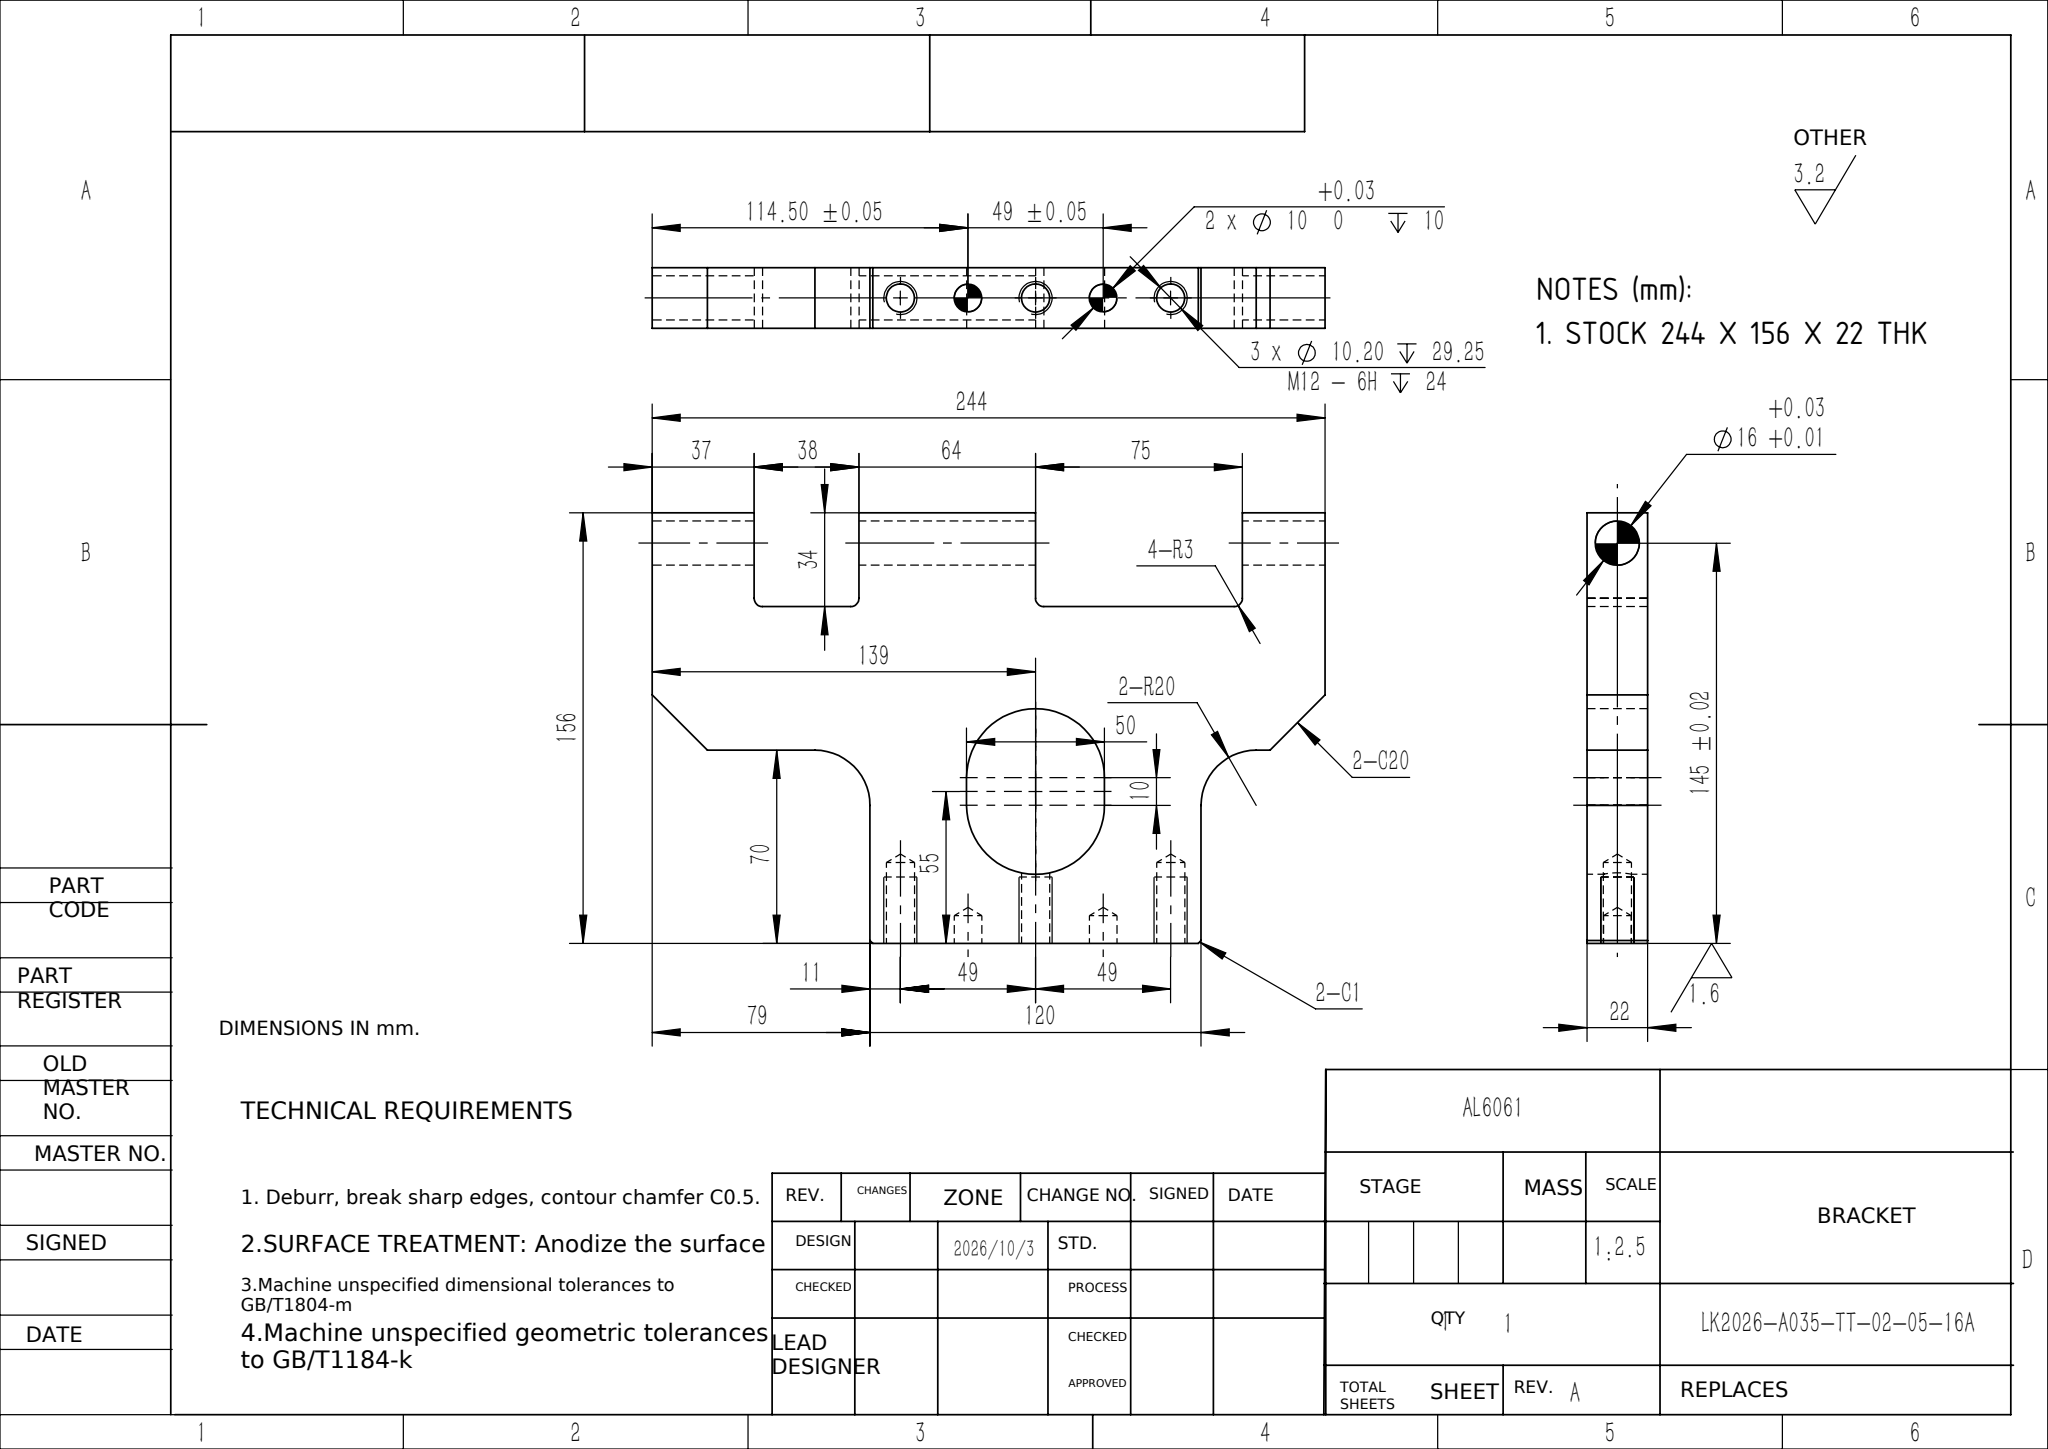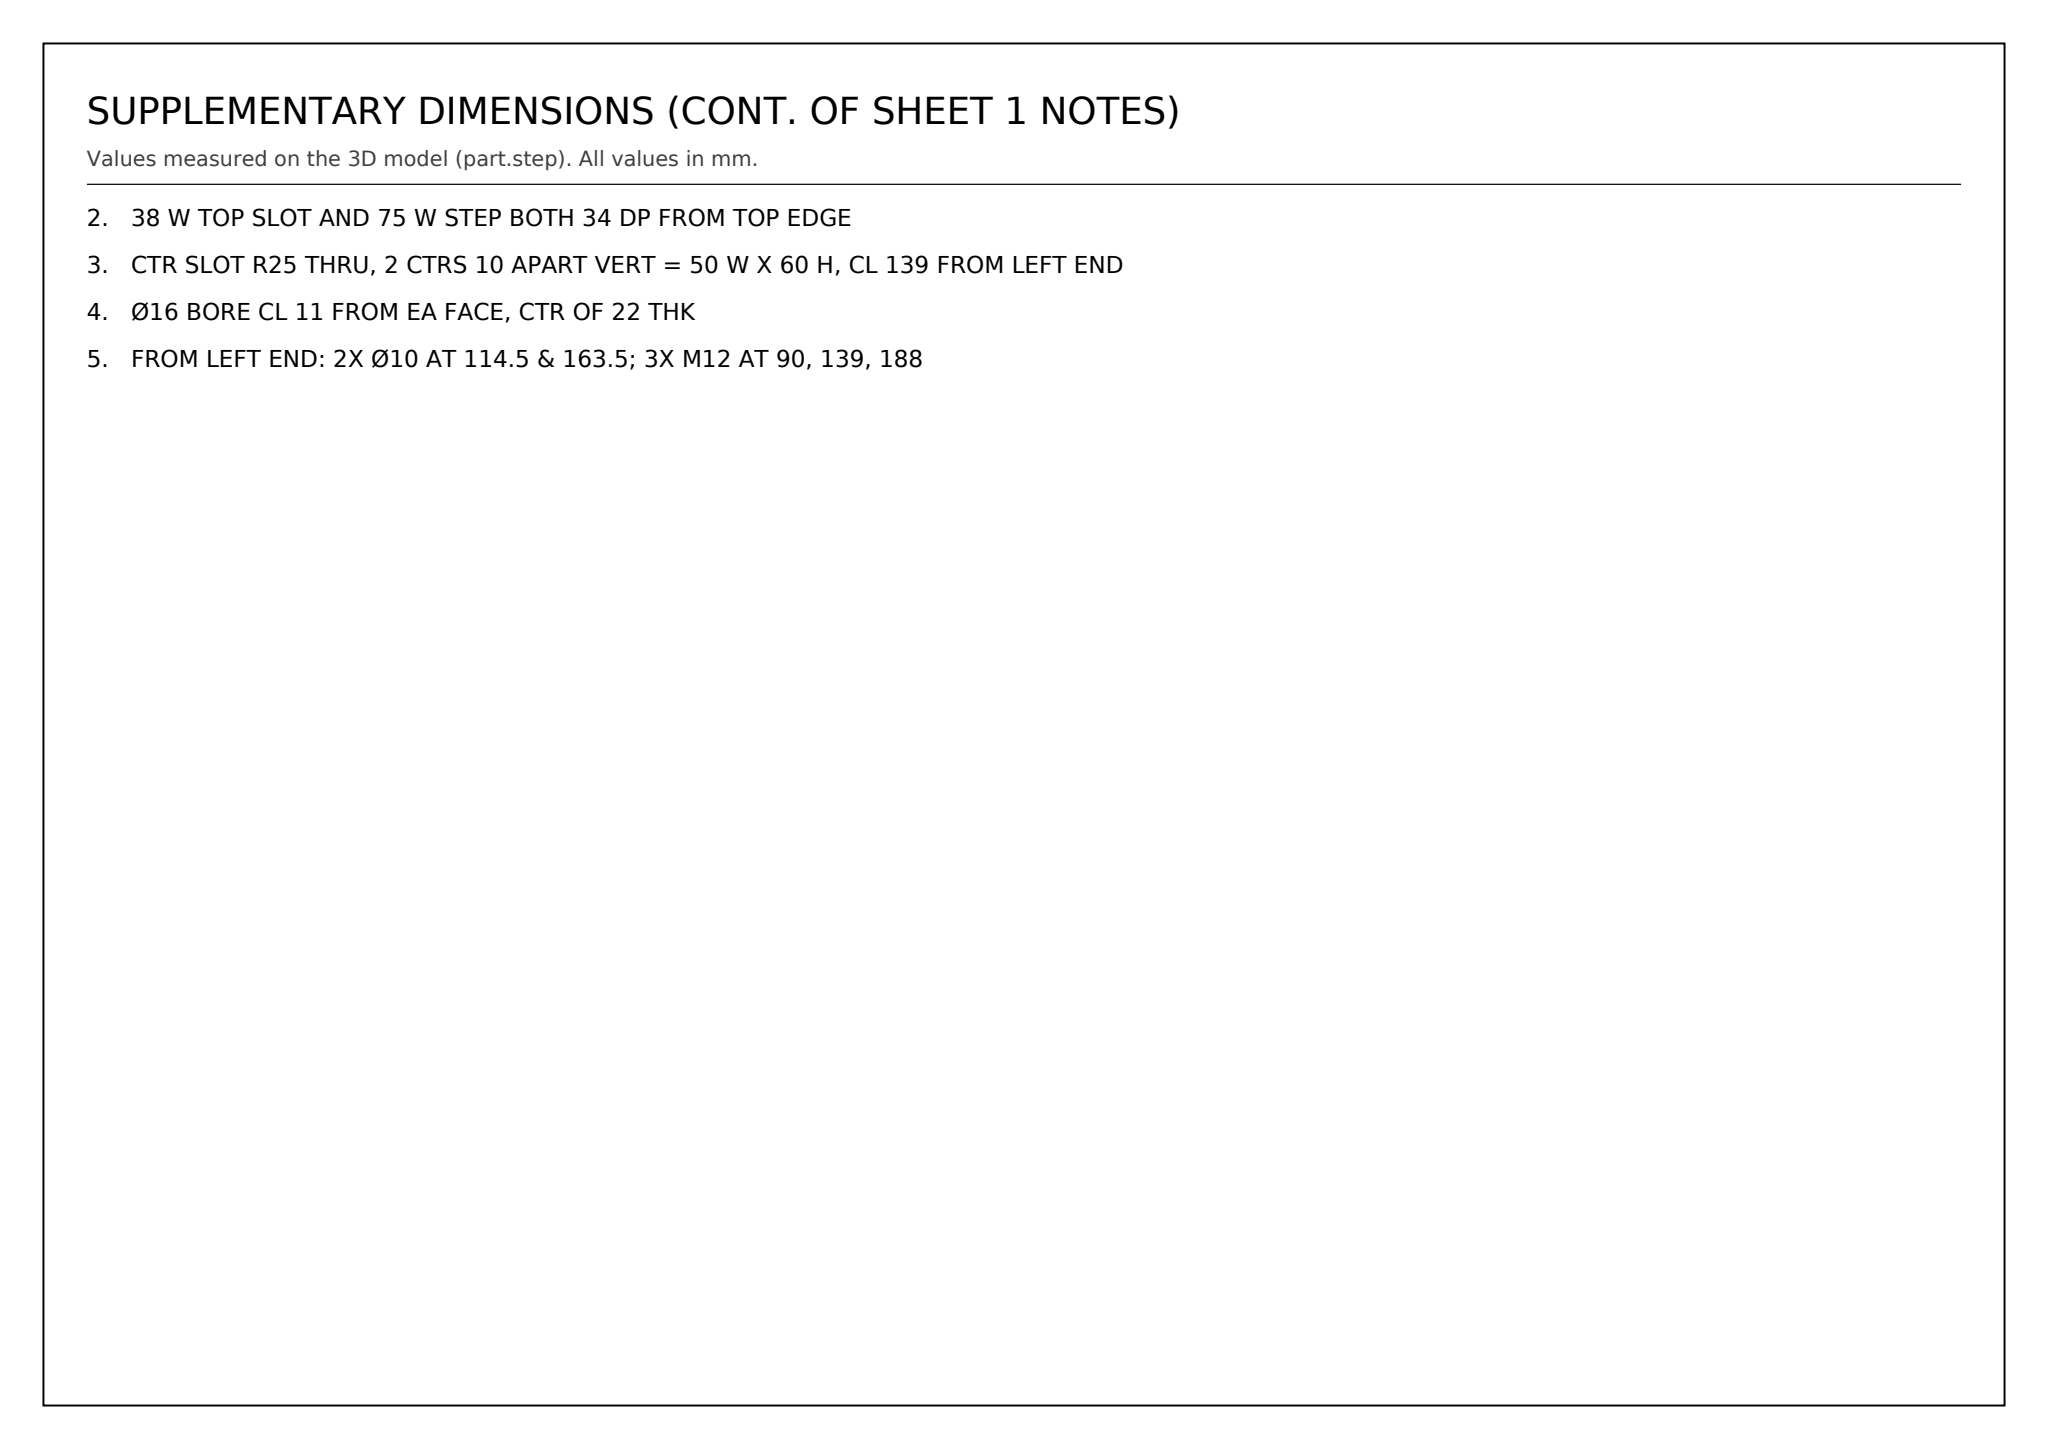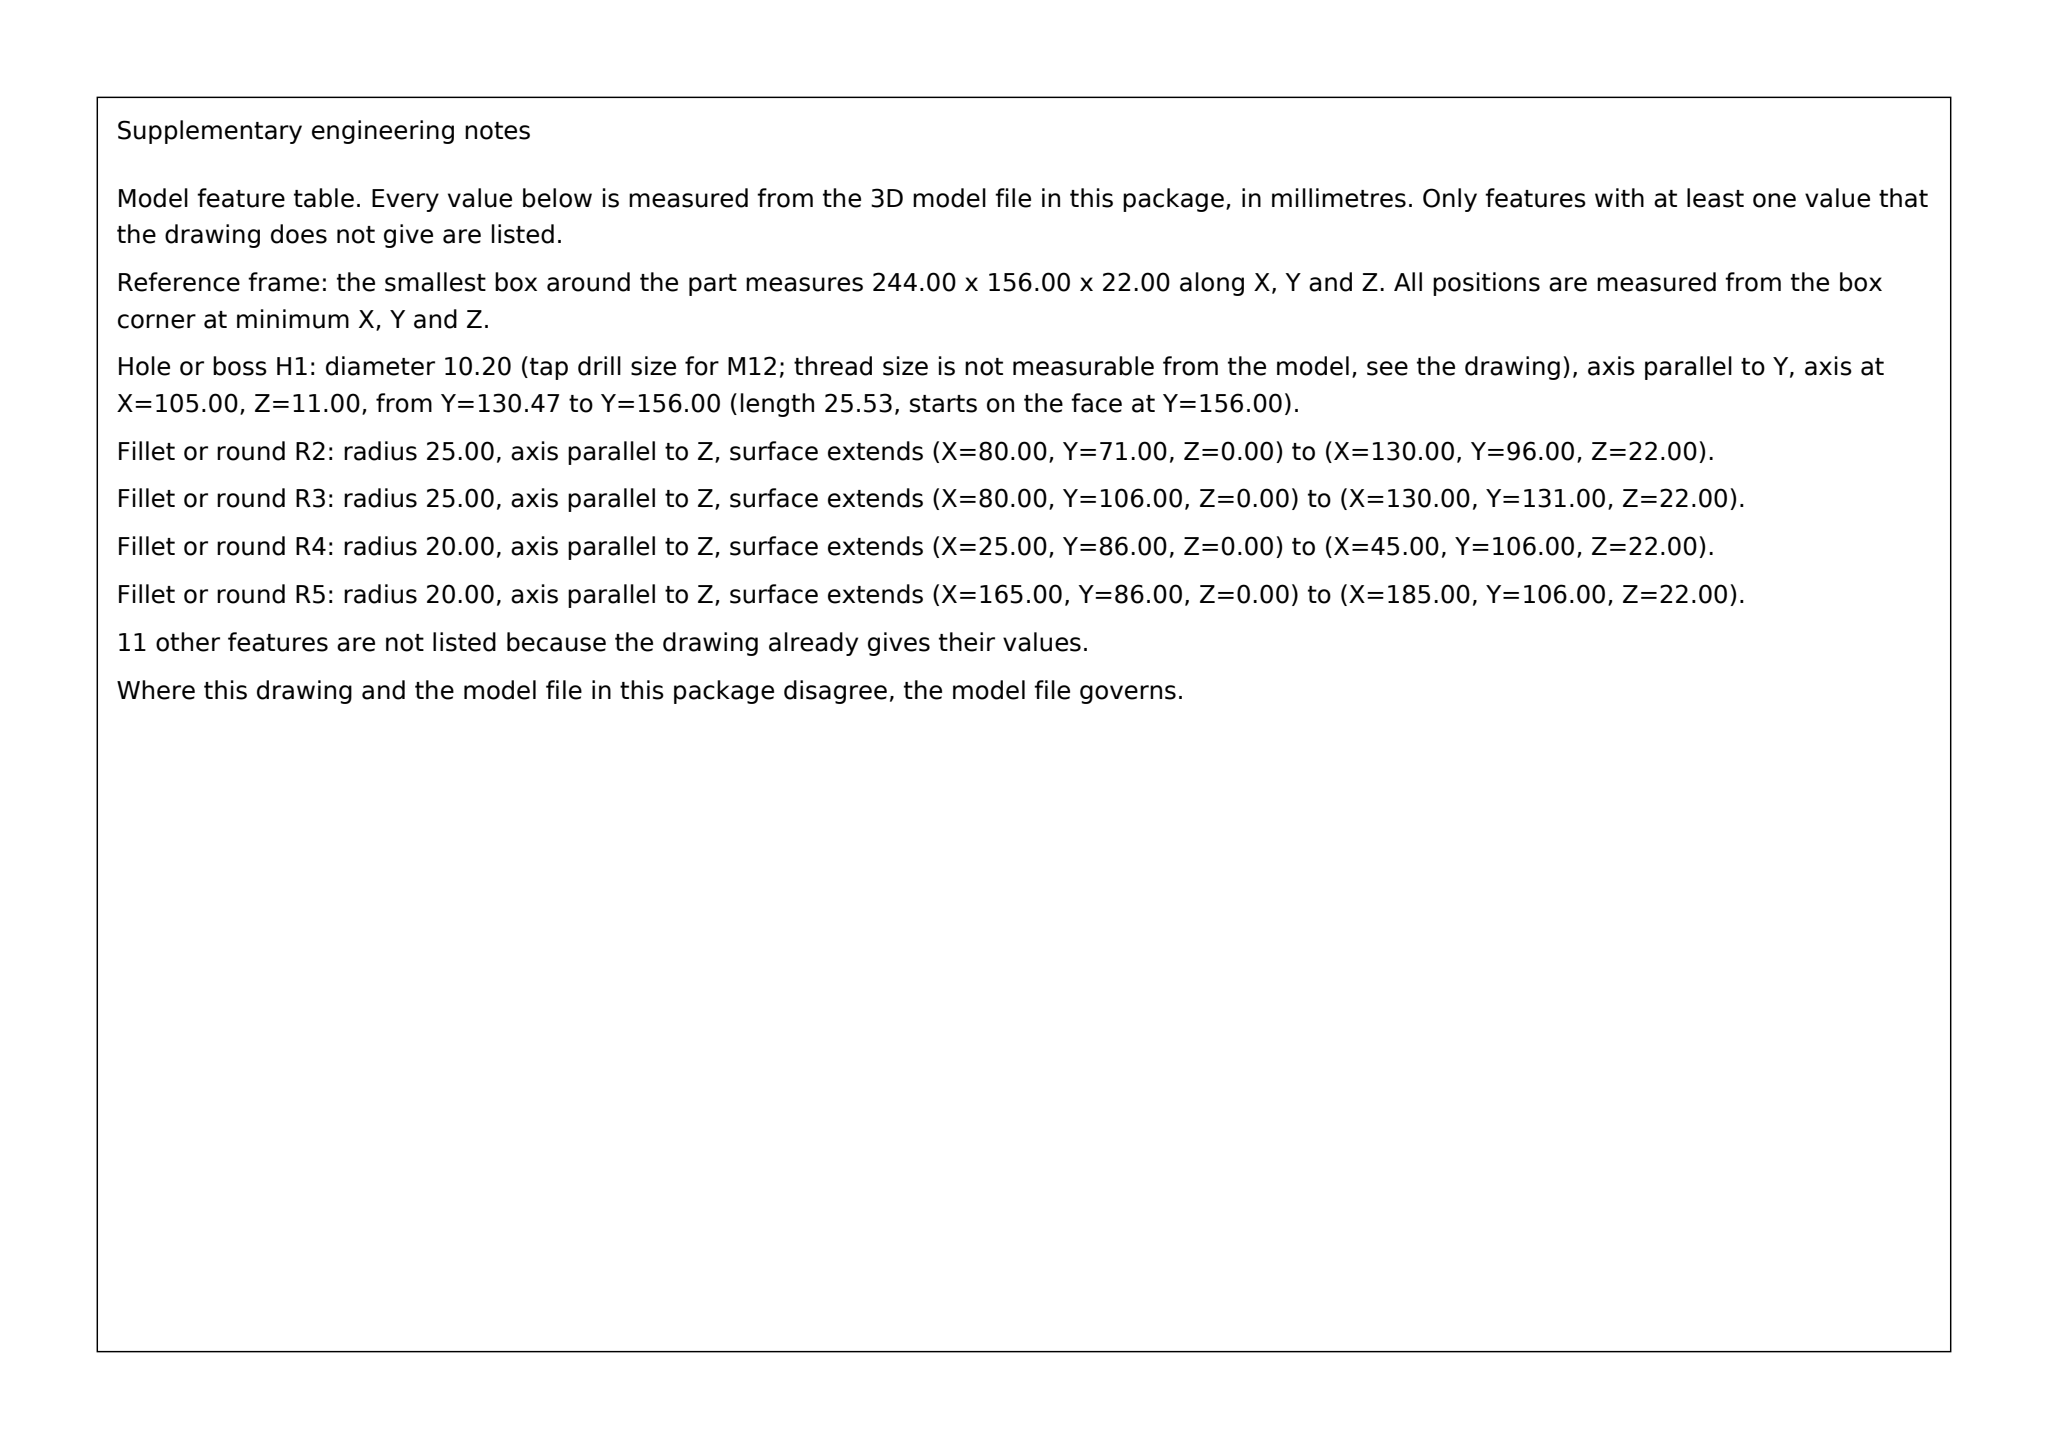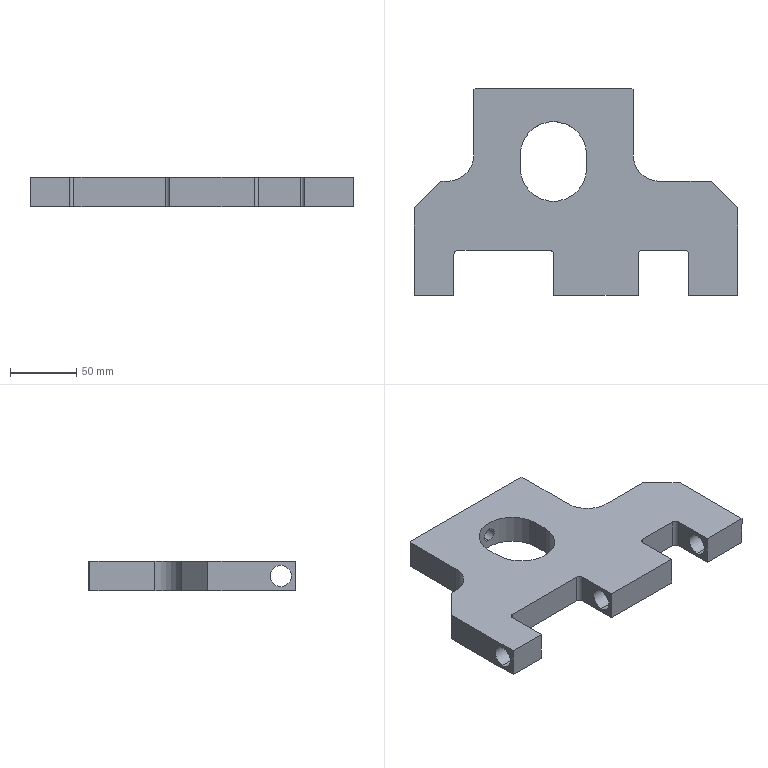Part | SolidWorks | mm | 1 solid | 56 faces | box 244 x 156 x 22 mm | volume 467785 mm3 | cylinder 24 | plane 24 | cone 8 | commonest cylinder face diameters 10.2 x6 16 x6 10 x4 6 x4 50 x2 40 x2
Drawing notes:
STOCK 244 X 156 X 22 THK | from the solid: bbox_xyz 244 x 156 x 22; z planes at 0 and 22
38 W TOP SLOT AND 75 W STEP BOTH 34 DP FROM TOP EDGE | from the solid: y planes at 34 (count 2) vs top face of 156 bbox -> both floors 34 from top edge
CTR SLOT R25 THRU, 2 CTRS 10 APART VERT = 50 W X 60 H, CL 139 FROM LEFT END | from the solid: Two Ø50 z-cylinders full 22 length at (105,96) and (105,106) -> obround 50 x 60, CL x=105
Ø16 BORE CL 11 FROM EA FACE, CTR OF 22 THK | from the solid: Ø16 x-axis bore at y=11, z=11; thickness planes z=0/z=22 -> CL centered, 145 from opposite edge
FROM LEFT END: 2X Ø10 AT 114.5 & 163.5; 3X M12 AT 90, 139, 188 | from the solid: Ø10 y-holes at x=80.5,129.5; Ø10.2/M12 y-holes at x=56,105,154; bbox X=244, left end = x244
build123d program:
from build123d import *

# Parameters (mm, degrees)
SKETCH1_W                     = 244
SKETCH1_H                     = 156
BOSS_EXTRUDE1_DEPTH           = 22
SKETCH2_W                     = 45
SKETCH2_H                     = 70
SKETCH2_W_2                   = 79
SKETCH2_W_3                   = 75
SKETCH2_H_2                   = 34
SKETCH2_W_4                   = 38
CUT_EXTRUDE1_DEPTH            = 147.465
SIZE_MM_DOWEL_PIN_HOLE1_D     = 16
M12_TAPPED_HOLE1_D            = 10.2
M12_TAPPED_HOLE1_DEPTH        = 29.25
M12_TAPPED_HOLE1_TIP          = 3.064
SIZE_MM_DOWEL_PIN_HOLE2_D     = 10
SIZE_MM_DOWEL_PIN_HOLE2_DEPTH = 10
SIZE_MM_DOWEL_PIN_HOLE2_TIP   = 3.004
FILLET1_R                     = 20
CHAMFER1_SIZE                 = 20
CHAMFER2_SIZE                 = 1
FILLET3_R                     = 3


with BuildPart() as part:
    # Sketch1 → Boss-Extrude1 (new body)
    with BuildSketch(Plane.XY):
        Rectangle(SKETCH1_W, SKETCH1_H)
    extrude(amount=BOSS_EXTRUDE1_DEPTH)

    # Sketch2 → Cut-Extrude1 (cut, through all)
    with BuildSketch(Plane.XY.offset(22)):
        with Locations((-99.5, 43)):
            Rectangle(SKETCH2_W, SKETCH2_H)
        with Locations((82.5, 43)):
            Rectangle(SKETCH2_W_2, SKETCH2_H)
        with BuildLine():
            Line((-42, 18), (-42, 28))
            ThreePointArc((-42, 28), (-17, 53), (8, 28))
            Line((8, 28), (8, 18))
            ThreePointArc((8, 18), (-17, -7), (-42, 18))
        make_face()
        with Locations((-54.5, -61)):
            Rectangle(SKETCH2_W_3, SKETCH2_H_2)
        with Locations((66, -61)):
            Rectangle(SKETCH2_W_4, SKETCH2_H_2)
    extrude(amount=-CUT_EXTRUDE1_DEPTH, mode=Mode.SUBTRACT)

    # Size mm Dowel Pin Hole1 (through all)
    with Locations(Plane.ZY.offset(122)):
        with Locations((11, -67)):
            Hole(SIZE_MM_DOWEL_PIN_HOLE1_D / 2)

    # M12 Tapped Hole1
    with Locations(Plane(origin=(0, 78, 0), x_dir=(1, 0, 0), z_dir=(0, 1, 0))):
        with Locations((-66, -11), (-17, -11), (32, -11)):
            Hole(M12_TAPPED_HOLE1_D / 2, depth=M12_TAPPED_HOLE1_DEPTH)
            with Locations((0, 0, -(M12_TAPPED_HOLE1_DEPTH + M12_TAPPED_HOLE1_TIP / 2))):  # 118° drill point
                Cone(0, M12_TAPPED_HOLE1_D / 2, M12_TAPPED_HOLE1_TIP, mode=Mode.SUBTRACT)

    # Size mm Dowel Pin Hole2
    with Locations(Plane(origin=(0, 78, 0), x_dir=(1, 0, 0), z_dir=(0, 1, 0))):
        with Locations((-41.5, -11), (7.5, -11)):
            Hole(SIZE_MM_DOWEL_PIN_HOLE2_D / 2, depth=SIZE_MM_DOWEL_PIN_HOLE2_DEPTH)
            with Locations((0, 0, -(SIZE_MM_DOWEL_PIN_HOLE2_DEPTH + SIZE_MM_DOWEL_PIN_HOLE2_TIP / 2))):  # 118° drill point
                Cone(0, SIZE_MM_DOWEL_PIN_HOLE2_D / 2, SIZE_MM_DOWEL_PIN_HOLE2_TIP, mode=Mode.SUBTRACT)

    # Fillet1
    fillet1_edges = [part.edges().sort_by_distance(p)[0] for p in [
        (43, 8, 11),
        (-77, 8, 11),
    ]]
    fillet(fillet1_edges, radius=FILLET1_R)

    # Chamfer1
    chamfer1_edges = [part.edges().sort_by_distance(p)[0] for p in [
        (122, 8, 11),
        (-122, 8, 11),
    ]]
    chamfer(chamfer1_edges, length=CHAMFER1_SIZE)

    # Chamfer2
    chamfer2_edges = [part.edges().sort_by_distance(p)[0] for p in [
        (43, 78, 11),
        (-77, 78, 11),
    ]]
    chamfer(chamfer2_edges, length=CHAMFER2_SIZE)

    # Fillet3
    fillet3_edges = [part.edges().sort_by_distance(p)[0] for p in [
        (47, -44, 11),
        (85, -44, 11),
        (-92, -44, 11),
        (-17, -44, 11),
    ]]
    fillet(fillet3_edges, radius=FILLET3_R)


solid = part.part